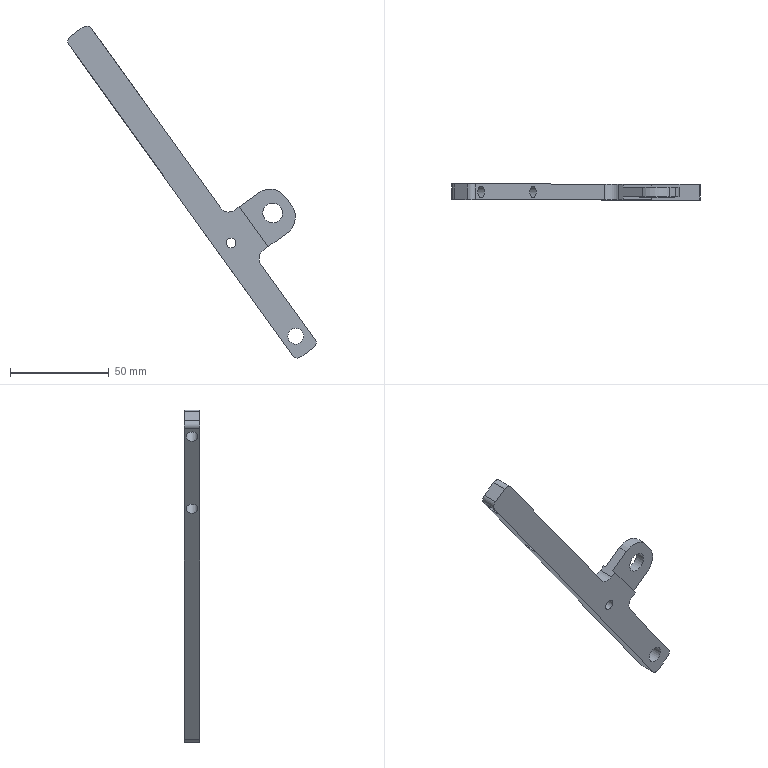Component | NX | CONNECTING_ROD | 1 solid | 27 faces | volume 24869 mm3 | plane 14 | cylinder 13 | commonest cylinder face diameters 6 x4 10 x3 20 x2 5.795 x2 8 x1 5 x1